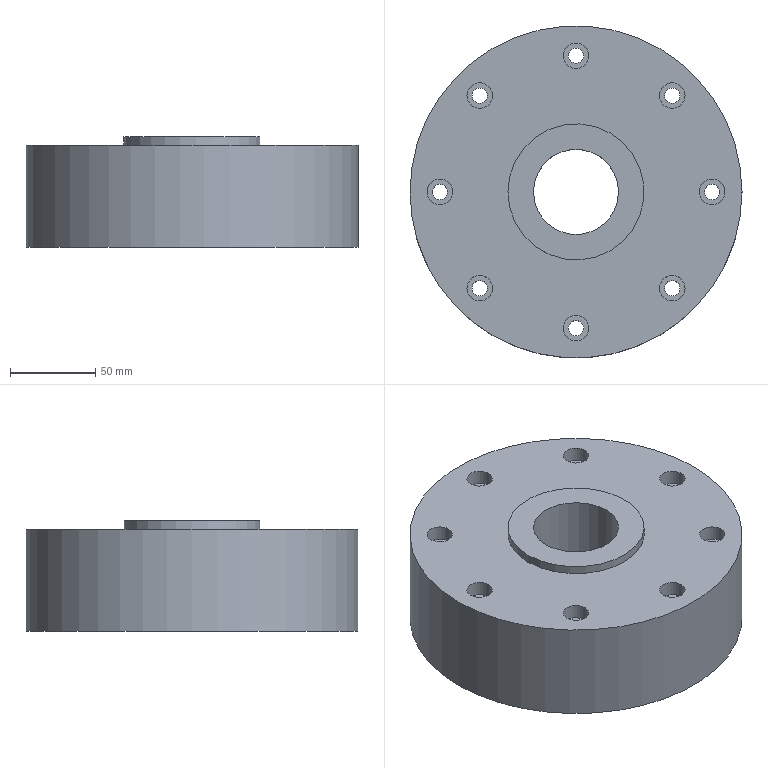Component | NX | FORCE_SENSOR | 1 solid | 31 faces | volume 1641992 mm3 | cylinder 19 | plane 11 | cone 1 | commonest cylinder face diameters 9 x8 15 x8 195 x1 50 x1 80 x1